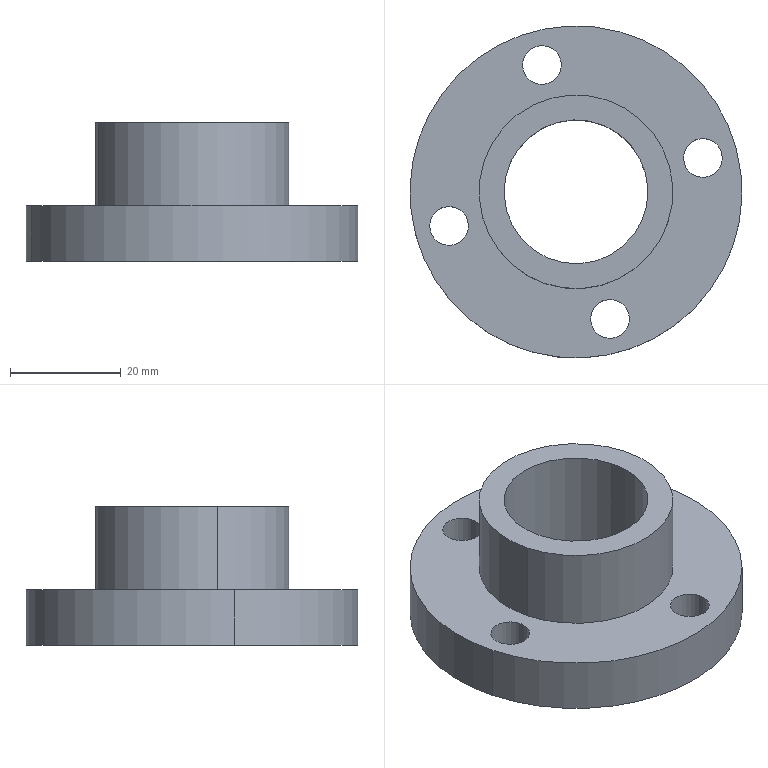Component | SolidWorks | SpindleFixtureAssemblyLeft-1_KLHFH011100CylinderConnectingSeatSLDPRT-1 | 1 solid | 17 faces | box 60 x 60 x 25 mm | volume 27893 mm3 | cylinder 14 | plane 3 | commonest cylinder face diameters 7 x8 26 x2 60 x2 35 x2 | material Plain Carbon Steel
STEP:
#1=COLOUR_RGB('',0.7922,0.8196,0.9333);
#2=FILL_AREA_STYLE_COLOUR('',#1);
#3=FILL_AREA_STYLE('',(#2));
#4=SURFACE_STYLE_FILL_AREA(#3);
#5=SURFACE_SIDE_STYLE('',(#4));
#6=SURFACE_STYLE_USAGE(.BOTH.,#5);
#7=PRESENTATION_STYLE_ASSIGNMENT((#6));
#8=CARTESIAN_POINT('',(0.4944,0.1325,-8.307));
#9=VERTEX_POINT('',#8);
#10=CARTESIAN_POINT('',(-0.4944,-0.1325,-8.307));
#11=VERTEX_POINT('',#10);
#12=CARTESIAN_POINT('',(0.,0.,-8.307));
#13=DIRECTION('',(0.,0.,1.));
#14=DIRECTION('',(-0.9659,-0.2588,0.));
#15=AXIS2_PLACEMENT_3D('',#12,#13,#14);
#16=CIRCLE('',#15,0.5118);
#17=EDGE_CURVE('',#9,#11,#16,.T.);
#18=ORIENTED_EDGE('',*,*,#17,.F.);
#19=CARTESIAN_POINT('',(0.4944,0.1325,-7.323));
#20=VERTEX_POINT('',#19);
#21=CARTESIAN_POINT('',(0.4944,0.1325,-7.323));
#22=DIRECTION('',(0.,0.,1.));
#23=VECTOR('',#22,39.37);
#24=LINE('',#21,#23);
#25=EDGE_CURVE('',#9,#20,#24,.T.);
#26=ORIENTED_EDGE('',*,*,#25,.T.);
#27=CARTESIAN_POINT('',(-0.4944,-0.1325,-7.323));
#28=VERTEX_POINT('',#27);
#29=CARTESIAN_POINT('',(0.,0.,-7.323));
#30=DIRECTION('',(0.,0.,1.));
#31=DIRECTION('',(-0.9659,-0.2588,0.));
#32=AXIS2_PLACEMENT_3D('',#29,#30,#31);
#33=CIRCLE('',#32,0.5118);
#34=EDGE_CURVE('',#20,#28,#33,.T.);
#35=ORIENTED_EDGE('',*,*,#34,.T.);
#36=CARTESIAN_POINT('',(-0.4944,-0.1325,-7.323));
#37=DIRECTION('',(0.,0.,1.));
#38=VECTOR('',#37,39.37);
#39=LINE('',#36,#38);
#40=EDGE_CURVE('',#11,#28,#39,.T.);
#41=ORIENTED_EDGE('',*,*,#40,.F.);
#42=EDGE_LOOP('',(#18,#26,#35,#41));
#43=FACE_OUTER_BOUND('',#42,.T.);
#44=CARTESIAN_POINT('',(0.,0.,-7.323));
#45=DIRECTION('',(0.,0.,1.));
#46=DIRECTION('',(-0.9659,-0.2588,0.));
#47=AXIS2_PLACEMENT_3D('',#44,#45,#46);
#48=CYLINDRICAL_SURFACE('',#47,0.5118);
#49=ADVANCED_FACE('',(#43),#48,.F.);
#50=CARTESIAN_POINT('',(0.3751,-0.8675,-8.307));
#51=VERTEX_POINT('',#50);
#52=CARTESIAN_POINT('',(0.1089,-0.9388,-8.307));
#53=VERTEX_POINT('',#52);
#54=CARTESIAN_POINT('',(0.242,-0.9032,-8.307));
#55=DIRECTION('',(0.,0.,1.));
#56=DIRECTION('',(-0.9659,-0.2588,0.));
#57=AXIS2_PLACEMENT_3D('',#54,#55,#56);
#58=CIRCLE('',#57,0.1378);
#59=EDGE_CURVE('',#51,#53,#58,.T.);
#60=ORIENTED_EDGE('',*,*,#59,.F.);
#61=CARTESIAN_POINT('',(0.3751,-0.8675,-7.913));
#62=VERTEX_POINT('',#61);
#63=CARTESIAN_POINT('',(0.3751,-0.8675,-7.913));
#64=DIRECTION('',(0.,0.,1.));
#65=VECTOR('',#64,39.37);
#66=LINE('',#63,#65);
#67=EDGE_CURVE('',#51,#62,#66,.T.);
#68=ORIENTED_EDGE('',*,*,#67,.T.);
#69=CARTESIAN_POINT('',(0.1089,-0.9388,-7.913));
#70=VERTEX_POINT('',#69);
#71=CARTESIAN_POINT('',(0.242,-0.9032,-7.913));
#72=DIRECTION('',(0.,0.,1.));
#73=DIRECTION('',(-0.9659,-0.2588,0.));
#74=AXIS2_PLACEMENT_3D('',#71,#72,#73);
#75=CIRCLE('',#74,0.1378);
#76=EDGE_CURVE('',#62,#70,#75,.T.);
#77=ORIENTED_EDGE('',*,*,#76,.T.);
#78=CARTESIAN_POINT('',(0.1089,-0.9388,-7.913));
#79=DIRECTION('',(0.,0.,1.));
#80=VECTOR('',#79,39.37);
#81=LINE('',#78,#80);
#82=EDGE_CURVE('',#53,#70,#81,.T.);
#83=ORIENTED_EDGE('',*,*,#82,.F.);
#84=EDGE_LOOP('',(#60,#68,#77,#83));
#85=FACE_OUTER_BOUND('',#84,.T.);
#86=CARTESIAN_POINT('',(0.242,-0.9032,-7.913));
#87=DIRECTION('',(0.,0.,1.));
#88=DIRECTION('',(-0.9659,-0.2588,0.));
#89=AXIS2_PLACEMENT_3D('',#86,#87,#88);
#90=CYLINDRICAL_SURFACE('',#89,0.1378);
#91=ADVANCED_FACE('',(#85),#90,.F.);
#92=CARTESIAN_POINT('',(-0.7701,-0.2063,-8.307));
#93=VERTEX_POINT('',#92);
#94=CARTESIAN_POINT('',(-1.036,-0.2777,-8.307));
#95=VERTEX_POINT('',#94);
#96=CARTESIAN_POINT('',(-0.9032,-0.242,-8.307));
#97=DIRECTION('',(0.,0.,1.));
#98=DIRECTION('',(-0.9659,-0.2588,0.));
#99=AXIS2_PLACEMENT_3D('',#96,#97,#98);
#100=CIRCLE('',#99,0.1378);
#101=EDGE_CURVE('',#93,#95,#100,.T.);
#102=ORIENTED_EDGE('',*,*,#101,.F.);
#103=CARTESIAN_POINT('',(-0.7701,-0.2063,-7.913));
#104=VERTEX_POINT('',#103);
#105=CARTESIAN_POINT('',(-0.7701,-0.2063,-7.913));
#106=DIRECTION('',(0.,0.,1.));
#107=VECTOR('',#106,39.37);
#108=LINE('',#105,#107);
#109=EDGE_CURVE('',#93,#104,#108,.T.);
#110=ORIENTED_EDGE('',*,*,#109,.T.);
#111=CARTESIAN_POINT('',(-1.036,-0.2777,-7.913));
#112=VERTEX_POINT('',#111);
#113=CARTESIAN_POINT('',(-0.9032,-0.242,-7.913));
#114=DIRECTION('',(0.,0.,1.));
#115=DIRECTION('',(-0.9659,-0.2588,0.));
#116=AXIS2_PLACEMENT_3D('',#113,#114,#115);
#117=CIRCLE('',#116,0.1378);
#118=EDGE_CURVE('',#104,#112,#117,.T.);
#119=ORIENTED_EDGE('',*,*,#118,.T.);
#120=CARTESIAN_POINT('',(-1.036,-0.2777,-7.913));
#121=DIRECTION('',(0.,0.,1.));
#122=VECTOR('',#121,39.37);
#123=LINE('',#120,#122);
#124=EDGE_CURVE('',#95,#112,#123,.T.);
#125=ORIENTED_EDGE('',*,*,#124,.F.);
#126=EDGE_LOOP('',(#102,#110,#119,#125));
#127=FACE_OUTER_BOUND('',#126,.T.);
#128=CARTESIAN_POINT('',(-0.9032,-0.242,-7.913));
#129=DIRECTION('',(0.,0.,1.));
#130=DIRECTION('',(-0.9659,-0.2588,0.));
#131=AXIS2_PLACEMENT_3D('',#128,#129,#130);
#132=CYLINDRICAL_SURFACE('',#131,0.1378);
#133=ADVANCED_FACE('',(#127),#132,.F.);
#134=CARTESIAN_POINT('',(-0.1089,0.9388,-8.307));
#135=VERTEX_POINT('',#134);
#136=CARTESIAN_POINT('',(-0.3751,0.8675,-8.307));
#137=VERTEX_POINT('',#136);
#138=CARTESIAN_POINT('',(-0.242,0.9032,-8.307));
#139=DIRECTION('',(0.,0.,1.));
#140=DIRECTION('',(-0.9659,-0.2588,0.));
#141=AXIS2_PLACEMENT_3D('',#138,#139,#140);
#142=CIRCLE('',#141,0.1378);
#143=EDGE_CURVE('',#135,#137,#142,.T.);
#144=ORIENTED_EDGE('',*,*,#143,.F.);
#145=CARTESIAN_POINT('',(-0.1089,0.9388,-7.913));
#146=VERTEX_POINT('',#145);
#147=CARTESIAN_POINT('',(-0.1089,0.9388,-7.913));
#148=DIRECTION('',(0.,0.,1.));
#149=VECTOR('',#148,39.37);
#150=LINE('',#147,#149);
#151=EDGE_CURVE('',#135,#146,#150,.T.);
#152=ORIENTED_EDGE('',*,*,#151,.T.);
#153=CARTESIAN_POINT('',(-0.3751,0.8675,-7.913));
#154=VERTEX_POINT('',#153);
#155=CARTESIAN_POINT('',(-0.242,0.9032,-7.913));
#156=DIRECTION('',(0.,0.,1.));
#157=DIRECTION('',(-0.9659,-0.2588,0.));
#158=AXIS2_PLACEMENT_3D('',#155,#156,#157);
#159=CIRCLE('',#158,0.1378);
#160=EDGE_CURVE('',#146,#154,#159,.T.);
#161=ORIENTED_EDGE('',*,*,#160,.T.);
#162=CARTESIAN_POINT('',(-0.3751,0.8675,-7.913));
#163=DIRECTION('',(0.,0.,1.));
#164=VECTOR('',#163,39.37);
#165=LINE('',#162,#164);
#166=EDGE_CURVE('',#137,#154,#165,.T.);
#167=ORIENTED_EDGE('',*,*,#166,.F.);
#168=EDGE_LOOP('',(#144,#152,#161,#167));
#169=FACE_OUTER_BOUND('',#168,.T.);
#170=CARTESIAN_POINT('',(-0.242,0.9032,-7.913));
#171=DIRECTION('',(0.,0.,1.));
#172=DIRECTION('',(-0.9659,-0.2588,0.));
#173=AXIS2_PLACEMENT_3D('',#170,#171,#172);
#174=CYLINDRICAL_SURFACE('',#173,0.1378);
#175=ADVANCED_FACE('',(#169),#174,.F.);
#176=CARTESIAN_POINT('',(1.036,0.2777,-8.307));
#177=VERTEX_POINT('',#176);
#178=CARTESIAN_POINT('',(0.7701,0.2063,-8.307));
#179=VERTEX_POINT('',#178);
#180=CARTESIAN_POINT('',(0.9032,0.242,-8.307));
#181=DIRECTION('',(0.,0.,1.));
#182=DIRECTION('',(-0.9659,-0.2588,0.));
#183=AXIS2_PLACEMENT_3D('',#180,#181,#182);
#184=CIRCLE('',#183,0.1378);
#185=EDGE_CURVE('',#177,#179,#184,.T.);
#186=ORIENTED_EDGE('',*,*,#185,.F.);
#187=CARTESIAN_POINT('',(1.036,0.2777,-7.913));
#188=VERTEX_POINT('',#187);
#189=CARTESIAN_POINT('',(1.036,0.2777,-7.913));
#190=DIRECTION('',(0.,0.,1.));
#191=VECTOR('',#190,39.37);
#192=LINE('',#189,#191);
#193=EDGE_CURVE('',#177,#188,#192,.T.);
#194=ORIENTED_EDGE('',*,*,#193,.T.);
#195=CARTESIAN_POINT('',(0.7701,0.2063,-7.913));
#196=VERTEX_POINT('',#195);
#197=CARTESIAN_POINT('',(0.9032,0.242,-7.913));
#198=DIRECTION('',(0.,0.,1.));
#199=DIRECTION('',(-0.9659,-0.2588,0.));
#200=AXIS2_PLACEMENT_3D('',#197,#198,#199);
#201=CIRCLE('',#200,0.1378);
#202=EDGE_CURVE('',#188,#196,#201,.T.);
#203=ORIENTED_EDGE('',*,*,#202,.T.);
#204=CARTESIAN_POINT('',(0.7701,0.2063,-7.913));
#205=DIRECTION('',(0.,0.,1.));
#206=VECTOR('',#205,39.37);
#207=LINE('',#204,#206);
#208=EDGE_CURVE('',#179,#196,#207,.T.);
#209=ORIENTED_EDGE('',*,*,#208,.F.);
#210=EDGE_LOOP('',(#186,#194,#203,#209));
#211=FACE_OUTER_BOUND('',#210,.T.);
#212=CARTESIAN_POINT('',(0.9032,0.242,-7.913));
#213=DIRECTION('',(0.,0.,1.));
#214=DIRECTION('',(-0.9659,-0.2588,0.));
#215=AXIS2_PLACEMENT_3D('',#212,#213,#214);
#216=CYLINDRICAL_SURFACE('',#215,0.1378);
#217=ADVANCED_FACE('',(#211),#216,.F.);
#218=CARTESIAN_POINT('',(1.141,0.3057,-8.307));
#219=VERTEX_POINT('',#218);
#220=CARTESIAN_POINT('',(-1.141,-0.3057,-8.307));
#221=VERTEX_POINT('',#220);
#222=CARTESIAN_POINT('',(0.,0.,-8.307));
#223=DIRECTION('',(0.,0.,-1.));
#224=DIRECTION('',(0.9659,0.2588,0.));
#225=AXIS2_PLACEMENT_3D('',#222,#223,#224);
#226=CIRCLE('',#225,1.181);
#227=EDGE_CURVE('',#219,#221,#226,.T.);
#228=ORIENTED_EDGE('',*,*,#227,.F.);
#229=CARTESIAN_POINT('',(1.141,0.3057,-7.913));
#230=VERTEX_POINT('',#229);
#231=CARTESIAN_POINT('',(1.141,0.3057,-8.307));
#232=DIRECTION('',(0.,0.,1.));
#233=VECTOR('',#232,39.37);
#234=LINE('',#231,#233);
#235=EDGE_CURVE('',#219,#230,#234,.T.);
#236=ORIENTED_EDGE('',*,*,#235,.T.);
#237=CARTESIAN_POINT('',(-1.141,-0.3057,-7.913));
#238=VERTEX_POINT('',#237);
#239=CARTESIAN_POINT('',(0.,0.,-7.913));
#240=DIRECTION('',(0.,0.,-1.));
#241=DIRECTION('',(0.9659,0.2588,0.));
#242=AXIS2_PLACEMENT_3D('',#239,#240,#241);
#243=CIRCLE('',#242,1.181);
#244=EDGE_CURVE('',#230,#238,#243,.T.);
#245=ORIENTED_EDGE('',*,*,#244,.T.);
#246=CARTESIAN_POINT('',(-1.141,-0.3057,-8.307));
#247=DIRECTION('',(0.,0.,1.));
#248=VECTOR('',#247,39.37);
#249=LINE('',#246,#248);
#250=EDGE_CURVE('',#221,#238,#249,.T.);
#251=ORIENTED_EDGE('',*,*,#250,.F.);
#252=EDGE_LOOP('',(#228,#236,#245,#251));
#253=FACE_OUTER_BOUND('',#252,.T.);
#254=CARTESIAN_POINT('',(0.,0.,-8.307));
#255=DIRECTION('',(0.,0.,1.));
#256=DIRECTION('',(-0.9659,-0.2588,0.));
#257=AXIS2_PLACEMENT_3D('',#254,#255,#256);
#258=CYLINDRICAL_SURFACE('',#257,1.181);
#259=ADVANCED_FACE('',(#253),#258,.T.);
#260=CARTESIAN_POINT('',(0.6655,0.1783,-7.913));
#261=VERTEX_POINT('',#260);
#262=CARTESIAN_POINT('',(-0.6655,-0.1783,-7.913));
#263=VERTEX_POINT('',#262);
#264=CARTESIAN_POINT('',(0.,0.,-7.913));
#265=DIRECTION('',(0.,0.,-1.));
#266=DIRECTION('',(0.9659,0.2588,0.));
#267=AXIS2_PLACEMENT_3D('',#264,#265,#266);
#268=CIRCLE('',#267,0.689);
#269=EDGE_CURVE('',#261,#263,#268,.T.);
#270=ORIENTED_EDGE('',*,*,#269,.F.);
#271=CARTESIAN_POINT('',(0.6655,0.1783,-7.323));
#272=VERTEX_POINT('',#271);
#273=CARTESIAN_POINT('',(0.6655,0.1783,-7.913));
#274=DIRECTION('',(0.,0.,1.));
#275=VECTOR('',#274,39.37);
#276=LINE('',#273,#275);
#277=EDGE_CURVE('',#261,#272,#276,.T.);
#278=ORIENTED_EDGE('',*,*,#277,.T.);
#279=CARTESIAN_POINT('',(-0.6655,-0.1783,-7.323));
#280=VERTEX_POINT('',#279);
#281=CARTESIAN_POINT('',(0.,0.,-7.323));
#282=DIRECTION('',(0.,0.,-1.));
#283=DIRECTION('',(0.9659,0.2588,0.));
#284=AXIS2_PLACEMENT_3D('',#281,#282,#283);
#285=CIRCLE('',#284,0.689);
#286=EDGE_CURVE('',#272,#280,#285,.T.);
#287=ORIENTED_EDGE('',*,*,#286,.T.);
#288=CARTESIAN_POINT('',(-0.6655,-0.1783,-7.913));
#289=DIRECTION('',(0.,0.,1.));
#290=VECTOR('',#289,39.37);
#291=LINE('',#288,#290);
#292=EDGE_CURVE('',#263,#280,#291,.T.);
#293=ORIENTED_EDGE('',*,*,#292,.F.);
#294=EDGE_LOOP('',(#270,#278,#287,#293));
#295=FACE_OUTER_BOUND('',#294,.T.);
#296=CARTESIAN_POINT('',(0.,0.,-7.913));
#297=DIRECTION('',(0.,0.,1.));
#298=DIRECTION('',(-0.9659,-0.2588,0.));
#299=AXIS2_PLACEMENT_3D('',#296,#297,#298);
#300=CYLINDRICAL_SURFACE('',#299,0.689);
#301=ADVANCED_FACE('',(#295),#300,.T.);
#302=CARTESIAN_POINT('',(0.,0.,-8.307));
#303=DIRECTION('',(0.,0.,1.));
#304=DIRECTION('',(-0.9659,-0.2588,0.));
#305=AXIS2_PLACEMENT_3D('',#302,#303,#304);
#306=CIRCLE('',#305,0.5118);
#307=EDGE_CURVE('',#11,#9,#306,.T.);
#308=ORIENTED_EDGE('',*,*,#307,.T.);
#309=ORIENTED_EDGE('',*,*,#17,.T.);
#310=EDGE_LOOP('',(#308,#309));
#311=FACE_BOUND('',#310,.T.);
#312=CARTESIAN_POINT('',(0.242,-0.9032,-8.307));
#313=DIRECTION('',(0.,0.,1.));
#314=DIRECTION('',(-0.9659,-0.2588,0.));
#315=AXIS2_PLACEMENT_3D('',#312,#313,#314);
#316=CIRCLE('',#315,0.1378);
#317=EDGE_CURVE('',#53,#51,#316,.T.);
#318=ORIENTED_EDGE('',*,*,#317,.T.);
#319=ORIENTED_EDGE('',*,*,#59,.T.);
#320=EDGE_LOOP('',(#318,#319));
#321=FACE_BOUND('',#320,.T.);
#322=CARTESIAN_POINT('',(-0.9032,-0.242,-8.307));
#323=DIRECTION('',(0.,0.,1.));
#324=DIRECTION('',(-0.9659,-0.2588,0.));
#325=AXIS2_PLACEMENT_3D('',#322,#323,#324);
#326=CIRCLE('',#325,0.1378);
#327=EDGE_CURVE('',#95,#93,#326,.T.);
#328=ORIENTED_EDGE('',*,*,#327,.T.);
#329=ORIENTED_EDGE('',*,*,#101,.T.);
#330=EDGE_LOOP('',(#328,#329));
#331=FACE_BOUND('',#330,.T.);
#332=CARTESIAN_POINT('',(-0.242,0.9032,-8.307));
#333=DIRECTION('',(0.,0.,1.));
#334=DIRECTION('',(-0.9659,-0.2588,0.));
#335=AXIS2_PLACEMENT_3D('',#332,#333,#334);
#336=CIRCLE('',#335,0.1378);
#337=EDGE_CURVE('',#137,#135,#336,.T.);
#338=ORIENTED_EDGE('',*,*,#337,.T.);
#339=ORIENTED_EDGE('',*,*,#143,.T.);
#340=EDGE_LOOP('',(#338,#339));
#341=FACE_BOUND('',#340,.T.);
#342=CARTESIAN_POINT('',(0.,0.,-8.307));
#343=DIRECTION('',(0.,0.,-1.));
#344=DIRECTION('',(0.9659,0.2588,0.));
#345=AXIS2_PLACEMENT_3D('',#342,#343,#344);
#346=CIRCLE('',#345,1.181);
#347=EDGE_CURVE('',#221,#219,#346,.T.);
#348=ORIENTED_EDGE('',*,*,#347,.T.);
#349=ORIENTED_EDGE('',*,*,#227,.T.);
#350=EDGE_LOOP('',(#348,#349));
#351=FACE_OUTER_BOUND('',#350,.T.);
#352=CARTESIAN_POINT('',(0.9032,0.242,-8.307));
#353=DIRECTION('',(0.,0.,1.));
#354=DIRECTION('',(-0.9659,-0.2588,0.));
#355=AXIS2_PLACEMENT_3D('',#352,#353,#354);
#356=CIRCLE('',#355,0.1378);
#357=EDGE_CURVE('',#179,#177,#356,.T.);
#358=ORIENTED_EDGE('',*,*,#357,.T.);
#359=ORIENTED_EDGE('',*,*,#185,.T.);
#360=EDGE_LOOP('',(#358,#359));
#361=FACE_BOUND('',#360,.T.);
#362=CARTESIAN_POINT('',(0.,0.,-8.307));
#363=DIRECTION('',(0.,0.,-1.));
#364=DIRECTION('',(0.9659,0.2588,0.));
#365=AXIS2_PLACEMENT_3D('',#362,#363,#364);
#366=PLANE('',#365);
#367=ADVANCED_FACE('',(#311,#321,#331,#341,#351,#361),#366,.T.);
#368=ORIENTED_EDGE('',*,*,#277,.F.);
#369=CARTESIAN_POINT('',(0.,0.,-7.913));
#370=DIRECTION('',(0.,0.,-1.));
#371=DIRECTION('',(0.9659,0.2588,0.));
#372=AXIS2_PLACEMENT_3D('',#369,#370,#371);
#373=CIRCLE('',#372,0.689);
#374=EDGE_CURVE('',#263,#261,#373,.T.);
#375=ORIENTED_EDGE('',*,*,#374,.F.);
#376=ORIENTED_EDGE('',*,*,#292,.T.);
#377=CARTESIAN_POINT('',(0.,0.,-7.323));
#378=DIRECTION('',(0.,0.,-1.));
#379=DIRECTION('',(0.9659,0.2588,0.));
#380=AXIS2_PLACEMENT_3D('',#377,#378,#379);
#381=CIRCLE('',#380,0.689);
#382=EDGE_CURVE('',#280,#272,#381,.T.);
#383=ORIENTED_EDGE('',*,*,#382,.T.);
#384=EDGE_LOOP('',(#368,#375,#376,#383));
#385=FACE_OUTER_BOUND('',#384,.T.);
#386=CARTESIAN_POINT('',(0.,0.,-7.913));
#387=DIRECTION('',(0.,0.,1.));
#388=DIRECTION('',(-0.9659,-0.2588,0.));
#389=AXIS2_PLACEMENT_3D('',#386,#387,#388);
#390=CYLINDRICAL_SURFACE('',#389,0.689);
#391=ADVANCED_FACE('',(#385),#390,.T.);
#392=CARTESIAN_POINT('',(0.,0.,-7.323));
#393=DIRECTION('',(0.,0.,1.));
#394=DIRECTION('',(-0.9659,-0.2588,0.));
#395=AXIS2_PLACEMENT_3D('',#392,#393,#394);
#396=CIRCLE('',#395,0.5118);
#397=EDGE_CURVE('',#28,#20,#396,.T.);
#398=ORIENTED_EDGE('',*,*,#397,.F.);
#399=ORIENTED_EDGE('',*,*,#34,.F.);
#400=EDGE_LOOP('',(#398,#399));
#401=FACE_BOUND('',#400,.T.);
#402=ORIENTED_EDGE('',*,*,#382,.F.);
#403=ORIENTED_EDGE('',*,*,#286,.F.);
#404=EDGE_LOOP('',(#402,#403));
#405=FACE_OUTER_BOUND('',#404,.T.);
#406=CARTESIAN_POINT('',(0.,0.,-7.323));
#407=DIRECTION('',(0.,0.,-1.));
#408=DIRECTION('',(0.9659,0.2588,0.));
#409=AXIS2_PLACEMENT_3D('',#406,#407,#408);
#410=PLANE('',#409);
#411=ADVANCED_FACE('',(#401,#405),#410,.F.);
#412=CARTESIAN_POINT('',(0.242,-0.9032,-7.913));
#413=DIRECTION('',(0.,0.,1.));
#414=DIRECTION('',(-0.9659,-0.2588,0.));
#415=AXIS2_PLACEMENT_3D('',#412,#413,#414);
#416=CIRCLE('',#415,0.1378);
#417=EDGE_CURVE('',#70,#62,#416,.T.);
#418=ORIENTED_EDGE('',*,*,#417,.F.);
#419=ORIENTED_EDGE('',*,*,#76,.F.);
#420=EDGE_LOOP('',(#418,#419));
#421=FACE_BOUND('',#420,.T.);
#422=CARTESIAN_POINT('',(-0.9032,-0.242,-7.913));
#423=DIRECTION('',(0.,0.,1.));
#424=DIRECTION('',(-0.9659,-0.2588,0.));
#425=AXIS2_PLACEMENT_3D('',#422,#423,#424);
#426=CIRCLE('',#425,0.1378);
#427=EDGE_CURVE('',#112,#104,#426,.T.);
#428=ORIENTED_EDGE('',*,*,#427,.F.);
#429=ORIENTED_EDGE('',*,*,#118,.F.);
#430=EDGE_LOOP('',(#428,#429));
#431=FACE_BOUND('',#430,.T.);
#432=CARTESIAN_POINT('',(-0.242,0.9032,-7.913));
#433=DIRECTION('',(0.,0.,1.));
#434=DIRECTION('',(-0.9659,-0.2588,0.));
#435=AXIS2_PLACEMENT_3D('',#432,#433,#434);
#436=CIRCLE('',#435,0.1378);
#437=EDGE_CURVE('',#154,#146,#436,.T.);
#438=ORIENTED_EDGE('',*,*,#437,.F.);
#439=ORIENTED_EDGE('',*,*,#160,.F.);
#440=EDGE_LOOP('',(#438,#439));
#441=FACE_BOUND('',#440,.T.);
#442=CARTESIAN_POINT('',(0.9032,0.242,-7.913));
#443=DIRECTION('',(0.,0.,1.));
#444=DIRECTION('',(-0.9659,-0.2588,0.));
#445=AXIS2_PLACEMENT_3D('',#442,#443,#444);
#446=CIRCLE('',#445,0.1378);
#447=EDGE_CURVE('',#196,#188,#446,.T.);
#448=ORIENTED_EDGE('',*,*,#447,.F.);
#449=ORIENTED_EDGE('',*,*,#202,.F.);
#450=EDGE_LOOP('',(#448,#449));
#451=FACE_BOUND('',#450,.T.);
#452=CARTESIAN_POINT('',(0.,0.,-7.913));
#453=DIRECTION('',(0.,0.,-1.));
#454=DIRECTION('',(0.9659,0.2588,0.));
#455=AXIS2_PLACEMENT_3D('',#452,#453,#454);
#456=CIRCLE('',#455,1.181);
#457=EDGE_CURVE('',#238,#230,#456,.T.);
#458=ORIENTED_EDGE('',*,*,#457,.F.);
#459=ORIENTED_EDGE('',*,*,#244,.F.);
#460=EDGE_LOOP('',(#458,#459));
#461=FACE_OUTER_BOUND('',#460,.T.);
#462=ORIENTED_EDGE('',*,*,#374,.T.);
#463=ORIENTED_EDGE('',*,*,#269,.T.);
#464=EDGE_LOOP('',(#462,#463));
#465=FACE_BOUND('',#464,.T.);
#466=CARTESIAN_POINT('',(0.,0.,-7.913));
#467=DIRECTION('',(0.,0.,-1.));
#468=DIRECTION('',(0.9659,0.2588,0.));
#469=AXIS2_PLACEMENT_3D('',#466,#467,#468);
#470=PLANE('',#469);
#471=ADVANCED_FACE('',(#421,#431,#441,#451,#461,#465),#470,.F.);
#472=ORIENTED_EDGE('',*,*,#235,.F.);
#473=ORIENTED_EDGE('',*,*,#347,.F.);
#474=ORIENTED_EDGE('',*,*,#250,.T.);
#475=ORIENTED_EDGE('',*,*,#457,.T.);
#476=EDGE_LOOP('',(#472,#473,#474,#475));
#477=FACE_OUTER_BOUND('',#476,.T.);
#478=CARTESIAN_POINT('',(0.,0.,-8.307));
#479=DIRECTION('',(0.,0.,1.));
#480=DIRECTION('',(-0.9659,-0.2588,0.));
#481=AXIS2_PLACEMENT_3D('',#478,#479,#480);
#482=CYLINDRICAL_SURFACE('',#481,1.181);
#483=ADVANCED_FACE('',(#477),#482,.T.);
#484=ORIENTED_EDGE('',*,*,#193,.F.);
#485=ORIENTED_EDGE('',*,*,#357,.F.);
#486=ORIENTED_EDGE('',*,*,#208,.T.);
#487=ORIENTED_EDGE('',*,*,#447,.T.);
#488=EDGE_LOOP('',(#484,#485,#486,#487));
#489=FACE_OUTER_BOUND('',#488,.T.);
#490=CARTESIAN_POINT('',(0.9032,0.242,-7.913));
#491=DIRECTION('',(0.,0.,1.));
#492=DIRECTION('',(-0.9659,-0.2588,0.));
#493=AXIS2_PLACEMENT_3D('',#490,#491,#492);
#494=CYLINDRICAL_SURFACE('',#493,0.1378);
#495=ADVANCED_FACE('',(#489),#494,.F.);
#496=ORIENTED_EDGE('',*,*,#151,.F.);
#497=ORIENTED_EDGE('',*,*,#337,.F.);
#498=ORIENTED_EDGE('',*,*,#166,.T.);
#499=ORIENTED_EDGE('',*,*,#437,.T.);
#500=EDGE_LOOP('',(#496,#497,#498,#499));
#501=FACE_OUTER_BOUND('',#500,.T.);
#502=CARTESIAN_POINT('',(-0.242,0.9032,-7.913));
#503=DIRECTION('',(0.,0.,1.));
#504=DIRECTION('',(-0.9659,-0.2588,0.));
#505=AXIS2_PLACEMENT_3D('',#502,#503,#504);
#506=CYLINDRICAL_SURFACE('',#505,0.1378);
#507=ADVANCED_FACE('',(#501),#506,.F.);
#508=ORIENTED_EDGE('',*,*,#109,.F.);
#509=ORIENTED_EDGE('',*,*,#327,.F.);
#510=ORIENTED_EDGE('',*,*,#124,.T.);
#511=ORIENTED_EDGE('',*,*,#427,.T.);
#512=EDGE_LOOP('',(#508,#509,#510,#511));
#513=FACE_OUTER_BOUND('',#512,.T.);
#514=CARTESIAN_POINT('',(-0.9032,-0.242,-7.913));
#515=DIRECTION('',(0.,0.,1.));
#516=DIRECTION('',(-0.9659,-0.2588,0.));
#517=AXIS2_PLACEMENT_3D('',#514,#515,#516);
#518=CYLINDRICAL_SURFACE('',#517,0.1378);
#519=ADVANCED_FACE('',(#513),#518,.F.);
#520=ORIENTED_EDGE('',*,*,#67,.F.);
#521=ORIENTED_EDGE('',*,*,#317,.F.);
#522=ORIENTED_EDGE('',*,*,#82,.T.);
#523=ORIENTED_EDGE('',*,*,#417,.T.);
#524=EDGE_LOOP('',(#520,#521,#522,#523));
#525=FACE_OUTER_BOUND('',#524,.T.);
#526=CARTESIAN_POINT('',(0.242,-0.9032,-7.913));
#527=DIRECTION('',(0.,0.,1.));
#528=DIRECTION('',(-0.9659,-0.2588,0.));
#529=AXIS2_PLACEMENT_3D('',#526,#527,#528);
#530=CYLINDRICAL_SURFACE('',#529,0.1378);
#531=ADVANCED_FACE('',(#525),#530,.F.);
#532=ORIENTED_EDGE('',*,*,#25,.F.);
#533=ORIENTED_EDGE('',*,*,#307,.F.);
#534=ORIENTED_EDGE('',*,*,#40,.T.);
#535=ORIENTED_EDGE('',*,*,#397,.T.);
#536=EDGE_LOOP('',(#532,#533,#534,#535));
#537=FACE_OUTER_BOUND('',#536,.T.);
#538=CARTESIAN_POINT('',(0.,0.,-7.323));
#539=DIRECTION('',(0.,0.,1.));
#540=DIRECTION('',(-0.9659,-0.2588,0.));
#541=AXIS2_PLACEMENT_3D('',#538,#539,#540);
#542=CYLINDRICAL_SURFACE('',#541,0.5118);
#543=ADVANCED_FACE('',(#537),#542,.F.);
#544=CLOSED_SHELL('',(#49,#91,#133,#175,#217,#259,#301,#367,#391,#411,#471,#483,#495,#507,#519,#531,#543));
#545=MANIFOLD_SOLID_BREP('',#544);
#546=STYLED_ITEM('',(#7),#545);
#547=PRESENTATION_LAYER_ASSIGNMENT('','',(#546));
#548=(LENGTH_UNIT()NAMED_UNIT(*)SI_UNIT($,.METRE.));
#549=LENGTH_MEASURE_WITH_UNIT(LENGTH_MEASURE(0.0254),#548);
#550=DIMENSIONAL_EXPONENTS(1.,0.,0.,0.,0.,0.,0.);
#551=(CONVERSION_BASED_UNIT('',#549)LENGTH_UNIT()NAMED_UNIT(#550));
#552=UNCERTAINTY_MEASURE_WITH_UNIT(LENGTH_MEASURE(0.00001),#551,'','');
#553=(NAMED_UNIT(*)PLANE_ANGLE_UNIT()SI_UNIT($,.RADIAN.));
#554=(NAMED_UNIT(*)SI_UNIT($,.STERADIAN.)SOLID_ANGLE_UNIT());
#555=(GEOMETRIC_REPRESENTATION_CONTEXT(3)GLOBAL_UNCERTAINTY_ASSIGNED_CONTEXT((#552))GLOBAL_UNIT_ASSIGNED_CONTEXT((#551,#553,#554))REPRESENTATION_CONTEXT('',''));
#556=MECHANICAL_DESIGN_GEOMETRIC_PRESENTATION_REPRESENTATION('',(#546),#555);
#557=CARTESIAN_POINT('',(0.,0.,0.));
#558=DIRECTION('',(0.,0.,1.));
#559=DIRECTION('',(1.,0.,0.));
#560=AXIS2_PLACEMENT_3D('',#557,#558,#559);
#561=(LENGTH_UNIT()NAMED_UNIT(*)SI_UNIT($,.METRE.));
#562=LENGTH_MEASURE_WITH_UNIT(LENGTH_MEASURE(0.0254),#561);
#563=DIMENSIONAL_EXPONENTS(1.,0.,0.,0.,0.,0.,0.);
#564=(CONVERSION_BASED_UNIT('',#562)LENGTH_UNIT()NAMED_UNIT(#563));
#565=UNCERTAINTY_MEASURE_WITH_UNIT(LENGTH_MEASURE(0.00001),#564,'','');
#566=(NAMED_UNIT(*)PLANE_ANGLE_UNIT()SI_UNIT($,.RADIAN.));
#567=(NAMED_UNIT(*)SI_UNIT($,.STERADIAN.)SOLID_ANGLE_UNIT());
#568=(GEOMETRIC_REPRESENTATION_CONTEXT(3)GLOBAL_UNCERTAINTY_ASSIGNED_CONTEXT((#565))GLOBAL_UNIT_ASSIGNED_CONTEXT((#564,#566,#567))REPRESENTATION_CONTEXT('',''));
#569=ADVANCED_BREP_SHAPE_REPRESENTATION('',(#545,#560),#568);